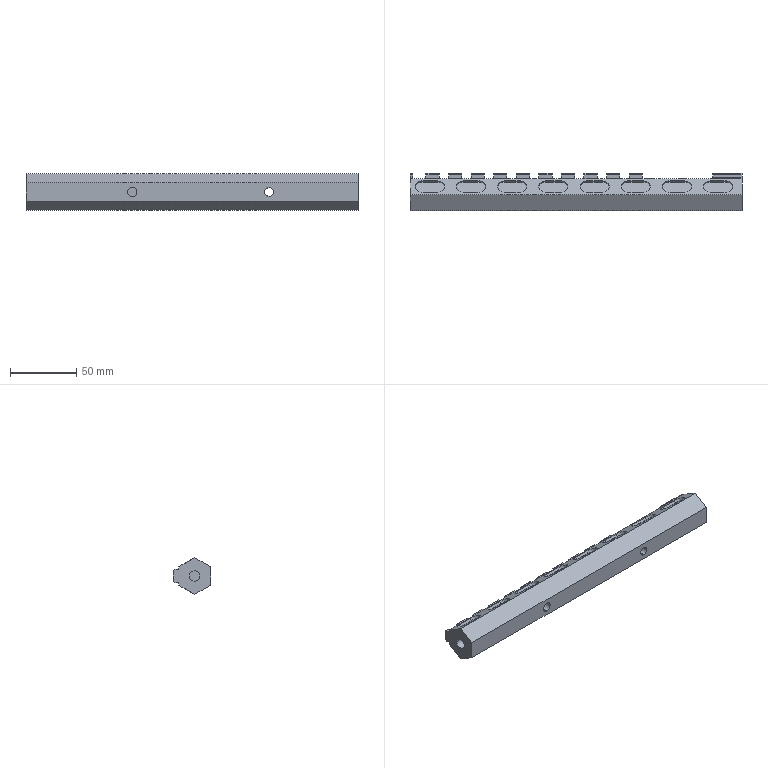Component | SolidWorks | UpperReceiver-1 | 1 solid | 198 faces | box 250 x 28 x 27.71 mm | volume 113722 mm3 | plane 145 | cylinder 50 | cone 3 | commonest cylinder face diameters 10 x34 6.5 x4 2 x3 7 x2 6 x2 12 x2 8 x2 18 x1